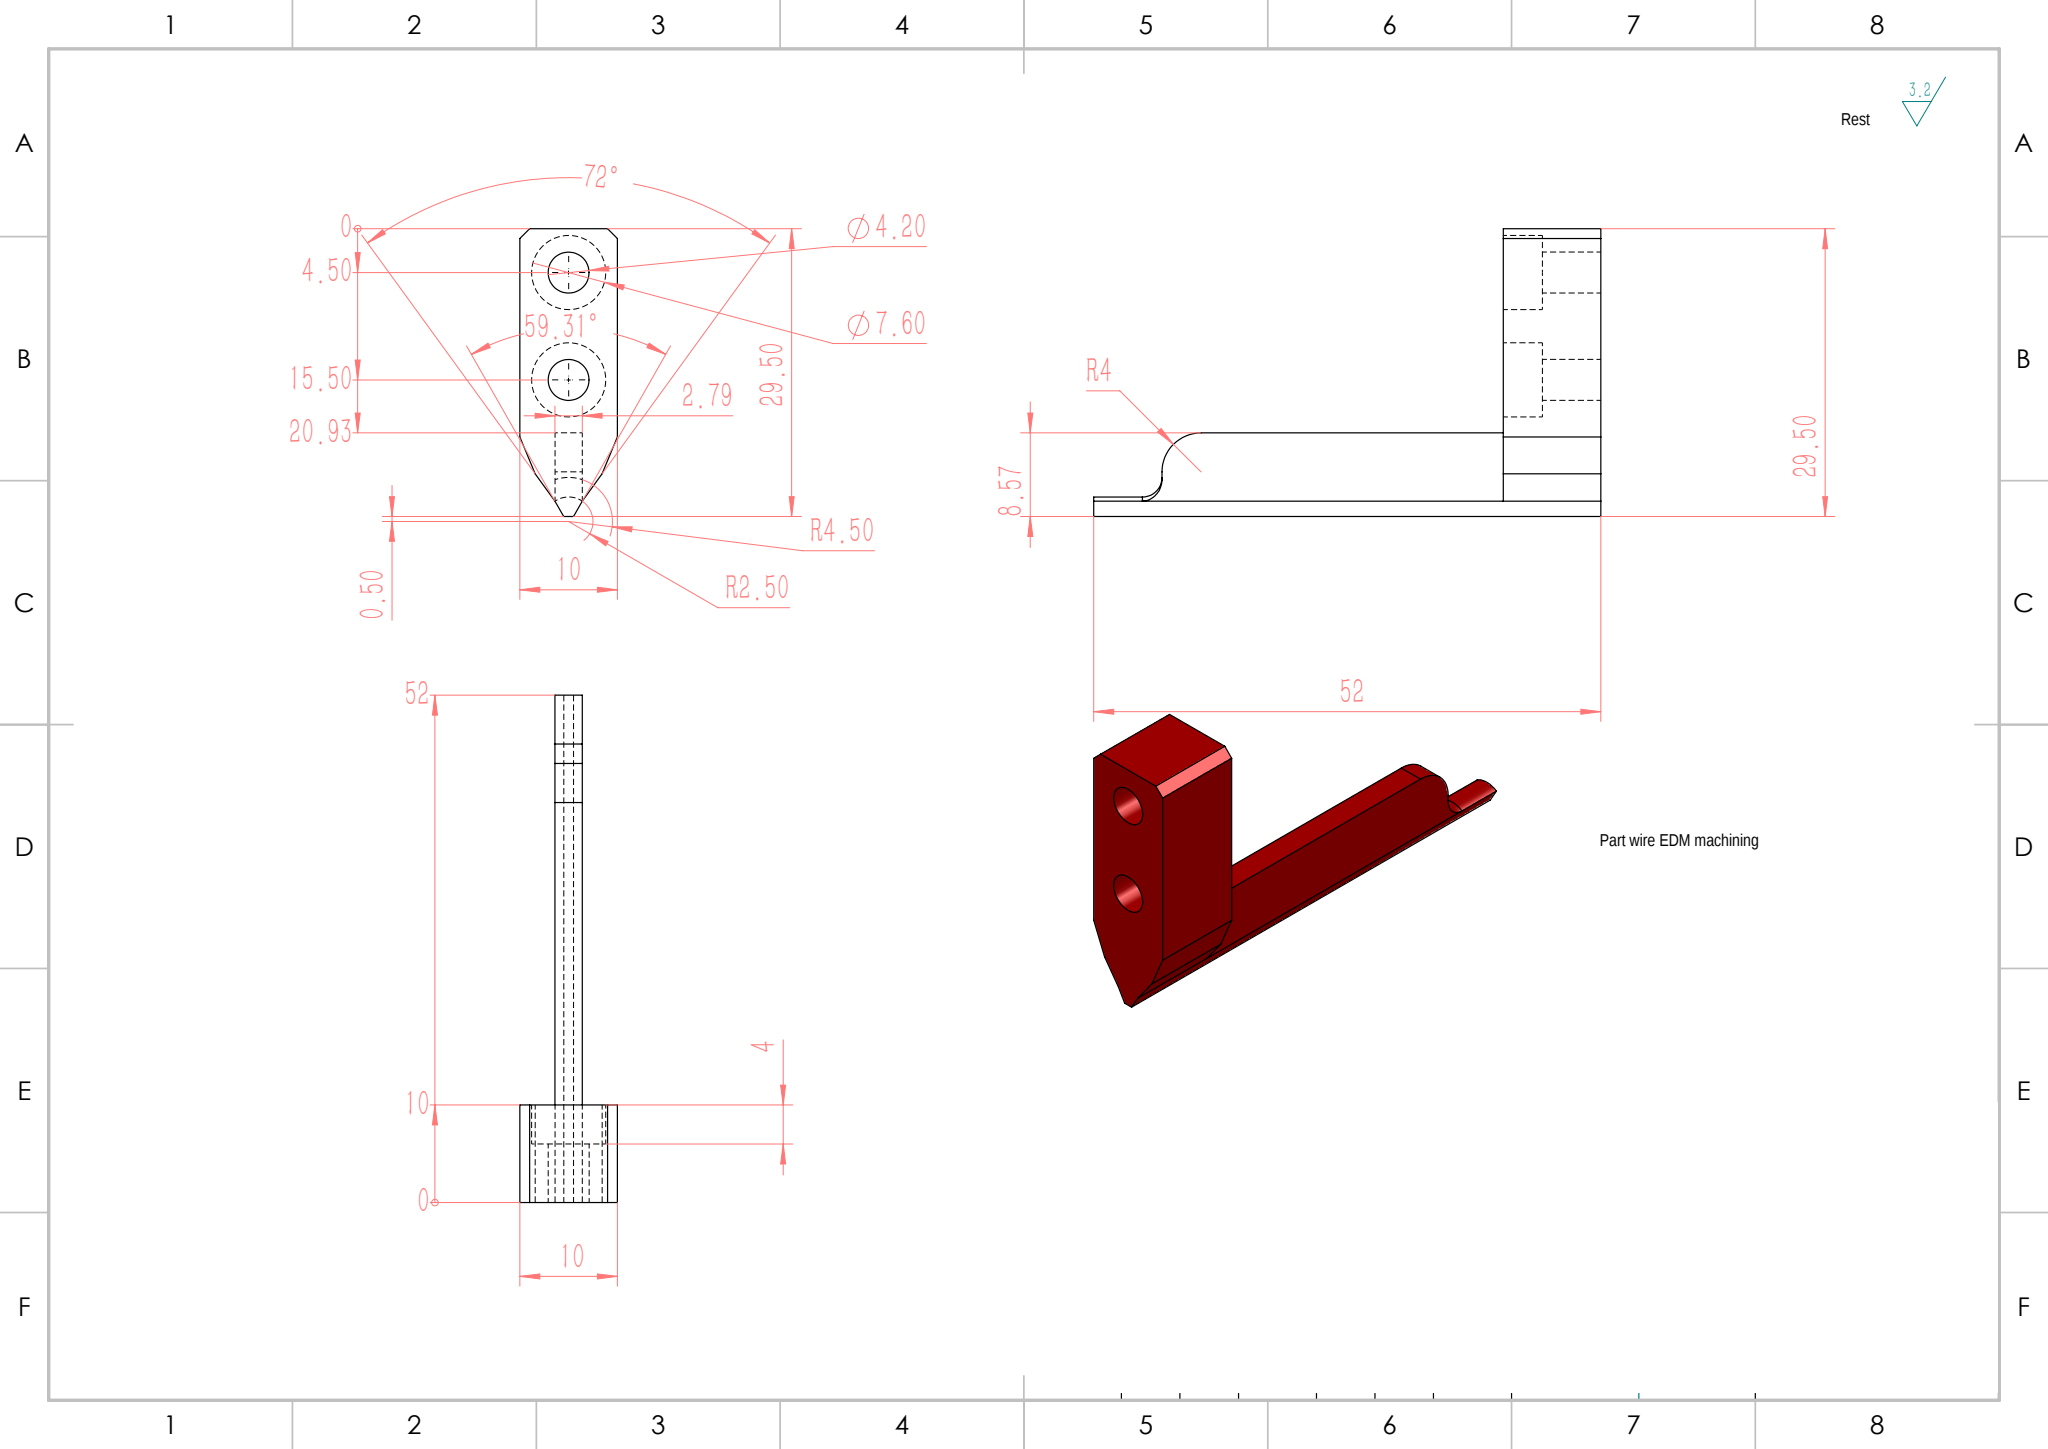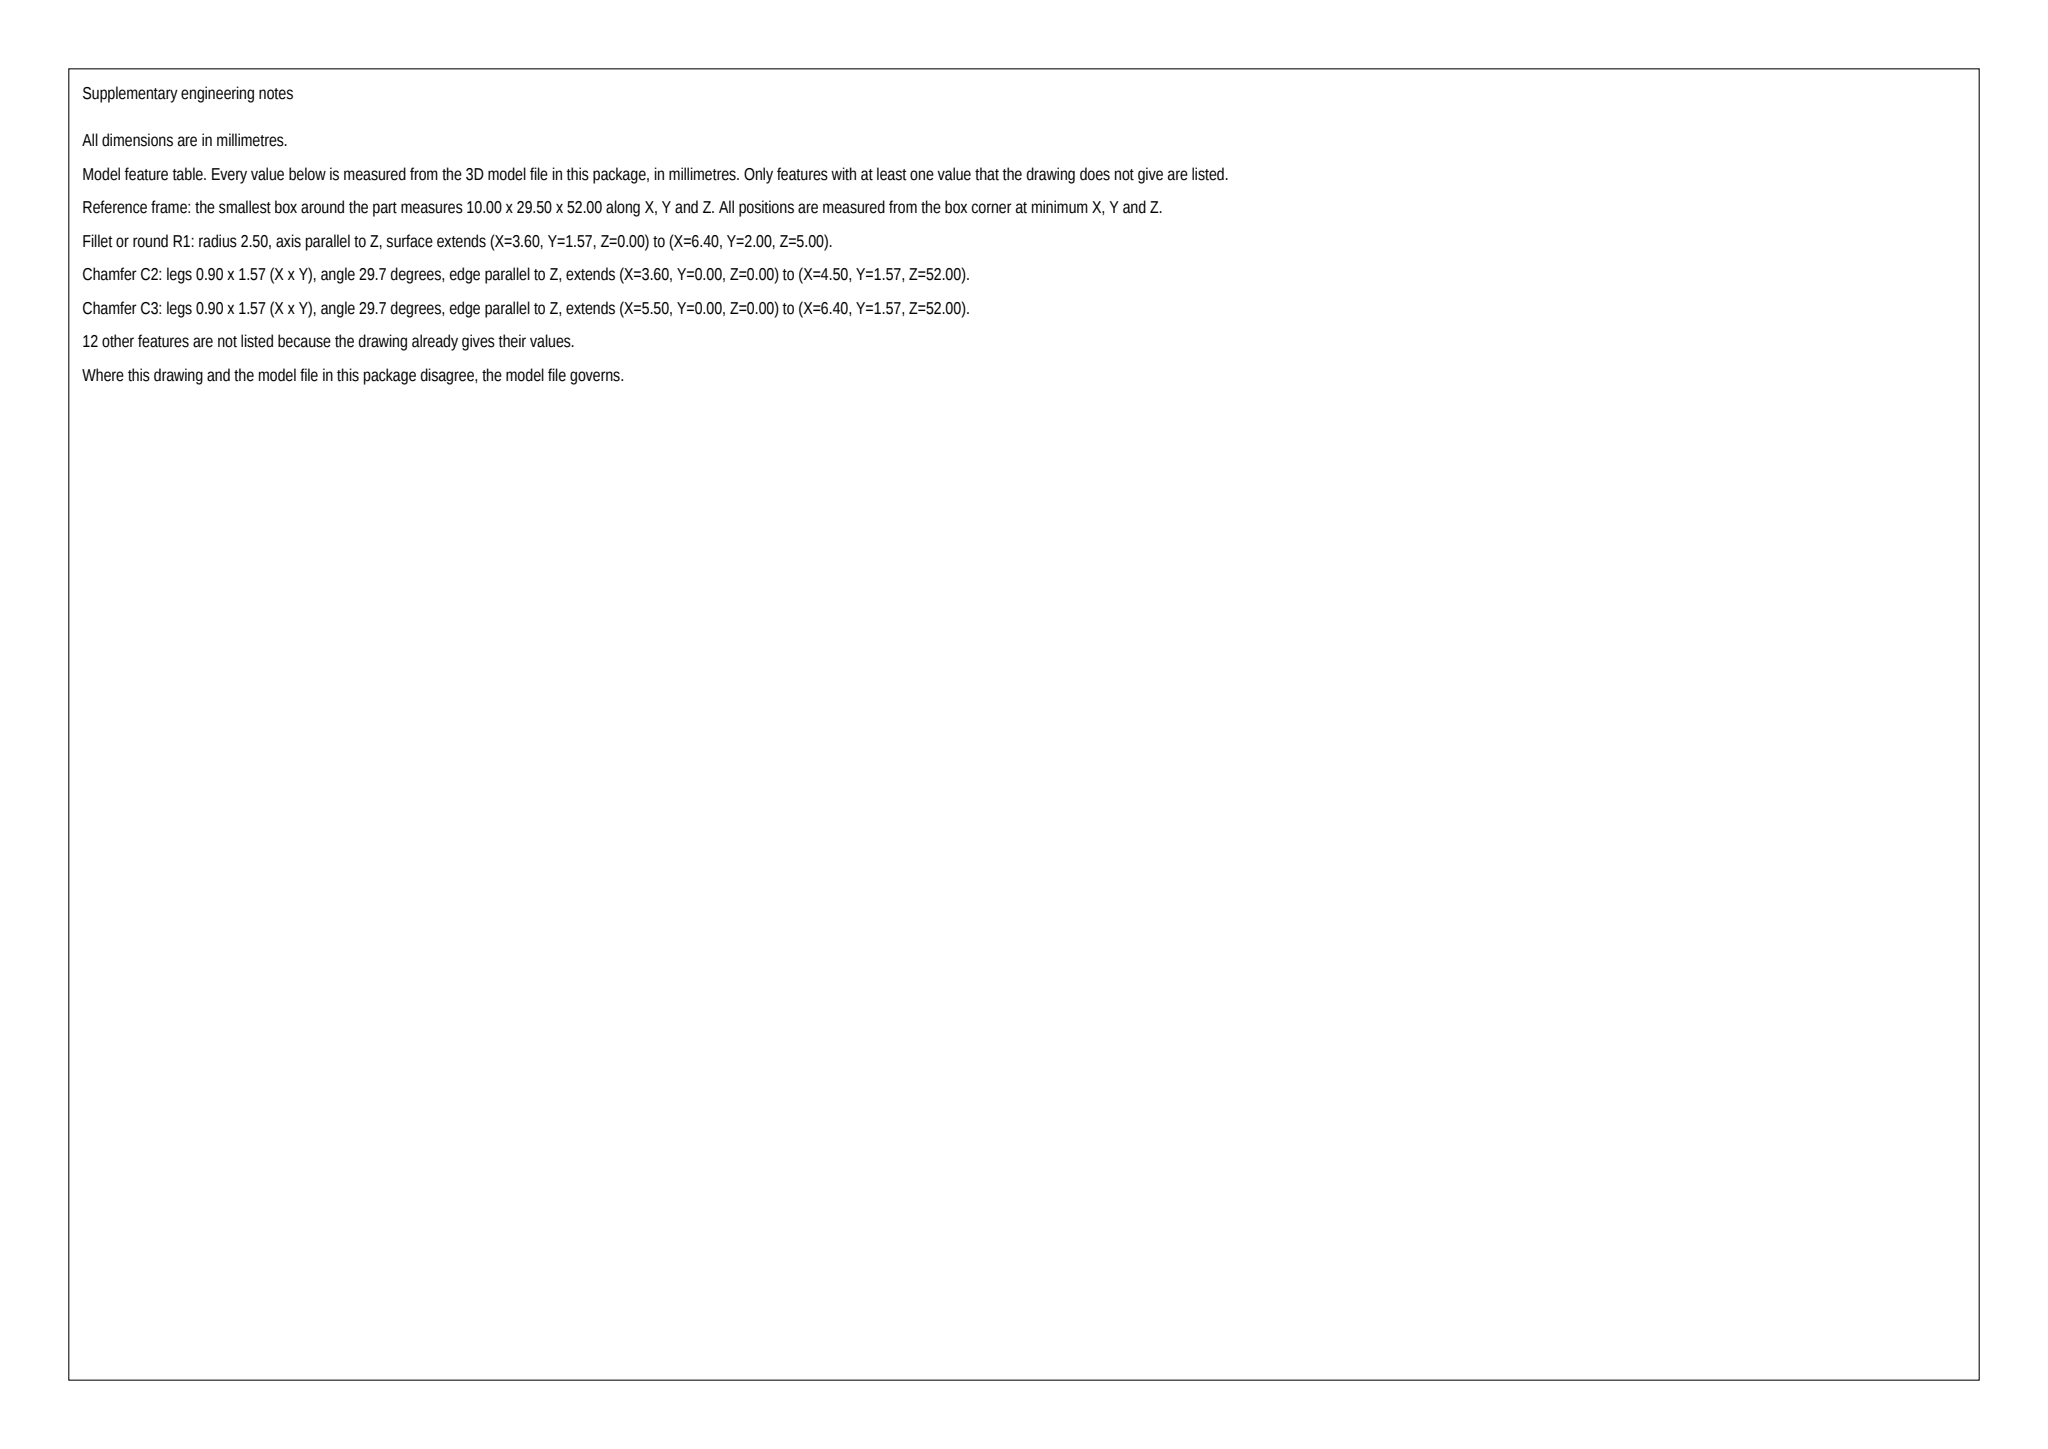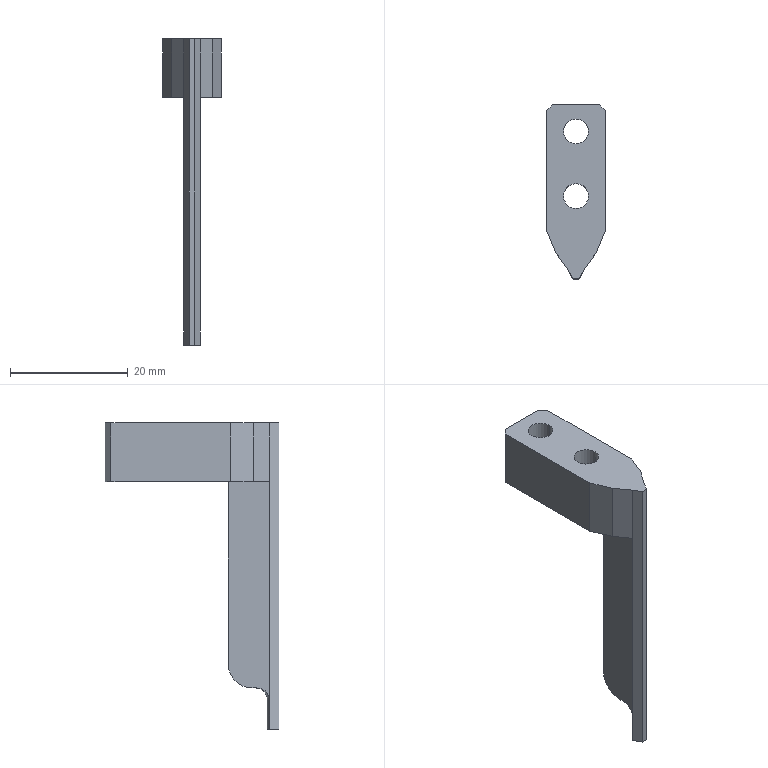Part | SolidWorks | mm | 1 solid | 32 faces | box 10 x 29.5 x 52 mm | volume 2887 mm3 | plane 21 | cylinder 10 | torus 1 | commonest cylinder face diameters 7.6 x4 4.2 x4 5 x1 8 x1
build123d program:
from build123d import *

# Parameters (mm, degrees)
SKETCH1_R                = 4.5
BOSS_EXTRUDE1_DEPTH      = 45
CHAMFER1_SIZE            = 3
CHAMFER1_SIZE2           = 8
SKETCH2_OUTSIDE_W        = 20.354
SKETCH2_OUTSIDE_H        = 20.354
CUT_EXTRUDE1_DEPTH       = 50
BOSS_EXTRUDE2_DEPTH      = 10
BOSS_EXTRUDE2_DEPTH_BACK = 30
BOSS_EXTRUDE3_DEPTH      = 40
SKETCH4_R                = 6.5
CUT_EXTRUDE2_DEPTH       = 60
CUT_EXTRUDE3_DEPTH       = 10
CUT_EXTRUDE3_DEPTH_BACK  = 30
SKETCH6_R                = 50
SKETCH6_R_2              = 10
SKETCH7_W                = 30.957
SKETCH7_H                = 17.267
CUT_EXTRUDE4_DEPTH       = 12.5
CHAMFER3_SIZE            = 1.732
CHAMFER3_SIZE2           = 3
SKETCH9_R                = 40
SKETCH9_R_2              = 30
CUT_EXTRUDE5_DEPTH       = 59.523
SKETCH11_R               = 2.1
CUT_EXTRUDE8_DEPTH       = 25
SKETCH12_W               = 21
SKETCH12_H               = 29
CUT_EXTRUDE9_DEPTH       = 51.249
BOSS_EXTRUDE4_DEPTH      = 10
BOSS_EXTRUDE6_START      = -52
BOSS_EXTRUDE6_DEPTH      = 52
BOSS_EXTRUDE7_START      = 35
BOSS_EXTRUDE7_DEPTH      = 35
FILLET1_R                = 2
SKETCH19_R               = 3.8
CUT_EXTRUDE10_DEPTH      = 4
FILLET2_R                = 4
SKETCH20_W               = 10
SKETCH20_H               = 0.4196
BOSS_EXTRUDE8_DEPTH      = 10
CHAMFER4_SIZE            = 1


with BuildPart() as part:
    # Sketch1 → Boss-Extrude1 (new body)
    with BuildSketch(Plane.XY):
        with Locations(Location((0, 0, 0), (0, 0, 180))):
            Circle(SKETCH1_R)
    extrude(amount=BOSS_EXTRUDE1_DEPTH)

    # Chamfer1
    chamfer1_edges = [part.edges().sort_by_distance(p)[0] for p in [
        (4.5, 0, 0),
    ]]
    chamfer1_side = [part.faces().sort_by_distance(p)[0] for p in [
        (0, 0, 0),
    ]]
    chamfer(chamfer1_edges, length=CHAMFER1_SIZE, length2=CHAMFER1_SIZE2, reference=chamfer1_side[0])

    # Sketch2 outside → Cut-Extrude1 (cut)
    with BuildSketch(Plane.XY.offset(45)):
        Rectangle(SKETCH2_OUTSIDE_W, SKETCH2_OUTSIDE_H)
        with BuildLine():
            Line((-3, 5.196), (0, 0))
            Line((0, 0), (3, 5.196))
            ThreePointArc((3, 5.196), (0, 6), (-3, 5.196))
        make_face(mode=Mode.SUBTRACT)
    extrude(amount=-CUT_EXTRUDE1_DEPTH, mode=Mode.SUBTRACT)

    # Sketch3 → Boss-Extrude2 (add, two sides: drawn at the far end of the back side and taken through both)
    with BuildSketch(Plane.XY.offset(45).offset(-BOSS_EXTRUDE2_DEPTH_BACK)):
        Polygon((-2.25, 3.897), (-2.25, 30), (2.25, 30), (2.25, 3.897), (0, 0), align=None)
    extrude(amount=BOSS_EXTRUDE2_DEPTH + BOSS_EXTRUDE2_DEPTH_BACK)

    # Sketch8 → Boss-Extrude3 (add)
    with BuildSketch(Plane.XY.offset(55)):
        Polygon((-5, 8.66), (0, 0), (5, 8.66), (5, 30), (-5, 30), align=None)
    extrude(amount=-BOSS_EXTRUDE3_DEPTH)

    # Sketch4 → Cut-Extrude2 (cut)
    with BuildSketch(Plane(origin=(0, 0, 0), x_dir=(-1, 0, 0), z_dir=(0, 0, -1))):
        with Locations((0, -4)):
            Circle(SKETCH4_R)
    extrude(amount=-CUT_EXTRUDE2_DEPTH, mode=Mode.SUBTRACT)

    # Sketch6 → Cut-Extrude3 (cut, two sides: drawn at the far end of the back side and taken through both)
    with BuildSketch(Plane(origin=(0, 0, 15), x_dir=(-1, 0, 0), z_dir=(0, 0, -1)).offset(-CUT_EXTRUDE3_DEPTH_BACK)):
        Circle(SKETCH6_R)
        Circle(SKETCH6_R_2, mode=Mode.SUBTRACT)
    extrude(amount=CUT_EXTRUDE3_DEPTH + CUT_EXTRUDE3_DEPTH_BACK, mode=Mode.SUBTRACT)

    # Sketch7 → Cut-Extrude4 (cut, symmetric)
    with BuildSketch(Plane(origin=(0, 0, 0), x_dir=(0, 0, -1), z_dir=(1, 0, 0))):
        with Locations((10.479, 0.9079)):
            Rectangle(SKETCH7_W, SKETCH7_H)
    extrude(amount=CUT_EXTRUDE4_DEPTH, both=True, mode=Mode.SUBTRACT)

    # Chamfer3
    chamfer3_edges = [part.edges().sort_by_distance(p)[0] for p in [
        (0, 10, 15),
    ]]
    chamfer3_side = [part.faces().sort_by_distance(p)[0] for p in [
        (0, 7.255, 15),
    ]]
    chamfer(chamfer3_edges, length=CHAMFER3_SIZE, length2=CHAMFER3_SIZE2, reference=chamfer3_side[0])

    # Sketch9 → Cut-Extrude5 (cut, through all)
    with BuildSketch(Plane(origin=(0, 0, 5), x_dir=(-1, 0, 0), z_dir=(0, 0, -1))):
        Circle(SKETCH9_R)
        Circle(SKETCH9_R_2, mode=Mode.SUBTRACT)
    extrude(amount=-CUT_EXTRUDE5_DEPTH, mode=Mode.SUBTRACT)

    # Sketch11 → Cut-Extrude8 (cut)
    with BuildSketch(Plane(origin=(0, 0, 45), x_dir=(-1, 0, 0), z_dir=(0, 0, -1))):
        with Locations((0, 25.5)):
            Circle(SKETCH11_R)
        with Locations((0, 14.5)):
            Circle(SKETCH11_R)
    extrude(amount=-CUT_EXTRUDE8_DEPTH, mode=Mode.SUBTRACT)

    # Sketch12 → Cut-Extrude9 (cut, through all)
    with BuildSketch(Plane(origin=(0, 0, 45), x_dir=(-1, 0, 0), z_dir=(0, 0, -1))):
        with Locations((0, 14.5)):
            Rectangle(SKETCH12_W, SKETCH12_H)
    extrude(amount=CUT_EXTRUDE9_DEPTH, mode=Mode.SUBTRACT)

    # Sketch13 → Boss-Extrude4 (add)
    with BuildSketch(Plane(origin=(0, 0, 45), x_dir=(-1, 0, 0), z_dir=(0, 0, -1))):
        with BuildLine():
            Line((5, 8.66), (-5, 8.66))
            Line((-5, 8.66), (-3.433, 4.878))
            Line((-3.433, 4.878), (-1.396, 2.074))
            ThreePointArc((-1.396, 2.074), (0, 2.5), (1.396, 2.074))
            Line((1.396, 2.074), (3.433, 4.878))
            Line((3.433, 4.878), (5, 8.66))
        make_face()
    extrude(amount=-BOSS_EXTRUDE4_DEPTH)

    # Sketch17 → Boss-Extrude6 (add)
    with BuildSketch(Plane.XY.offset(55).offset(BOSS_EXTRUDE6_START)):
        with BuildLine():
            Line((1.396, 2.074), (0.5, 0.5))
            Line((0.5, 0.5), (-0.5, 0.5))
            Line((-0.5, 0.5), (-1.396, 2.074))
            ThreePointArc((-1.396, 2.074), (0, 2.5), (1.396, 2.074))
        make_face()
    extrude(amount=BOSS_EXTRUDE6_DEPTH)

    # Sketch18 → Boss-Extrude7 (add)
    with BuildSketch(Plane(origin=(0, 0, 45), x_dir=(-1, 0, 0), z_dir=(0, 0, -1)).offset(BOSS_EXTRUDE7_START)):
        with BuildLine():
            Line((-1.396, 2.074), (-1.396, 9.074))
            Line((-1.396, 9.074), (1.396, 9.074))
            Line((1.396, 9.074), (1.396, 2.074))
            ThreePointArc((1.396, 2.074), (0, 2.5), (-1.396, 2.074))
        make_face()
    extrude(amount=-BOSS_EXTRUDE7_DEPTH)

    # Fillet1
    fillet1_edges = [part.edges().sort_by_distance(p)[0] for p in [
        (0, 2.5, 10),
    ]]
    fillet(fillet1_edges, radius=FILLET1_R)

    # Sketch19 → Cut-Extrude10 (cut)
    with BuildSketch(Plane(origin=(0, 0, 45), x_dir=(-1, 0, 0), z_dir=(0, 0, -1))):
        with Locations((0, 25.5)):
            Circle(SKETCH19_R)
        with Locations((0, 14.5)):
            Circle(SKETCH19_R)
    extrude(amount=-CUT_EXTRUDE10_DEPTH, mode=Mode.SUBTRACT)

    # Fillet2
    fillet2_edges = [part.edges().sort_by_distance(p)[0] for p in [
        (0, 9.074, 10),
    ]]
    fillet(fillet2_edges, radius=FILLET2_R)

    # Sketch20 → Boss-Extrude8 (add)
    with BuildSketch(Plane(origin=(0, 0, 45), x_dir=(-1, 0, 0), z_dir=(0, 0, -1))):
        with Locations((0, 29.79)):
            Rectangle(SKETCH20_W, SKETCH20_H)
    extrude(amount=-BOSS_EXTRUDE8_DEPTH)

    # Chamfer4
    chamfer4_edges = [part.edges().sort_by_distance(p)[0] for p in [
        (-5, 30, 50),
        (5, 30, 50),
    ]]
    chamfer(chamfer4_edges, length=CHAMFER4_SIZE)


solid = part.part